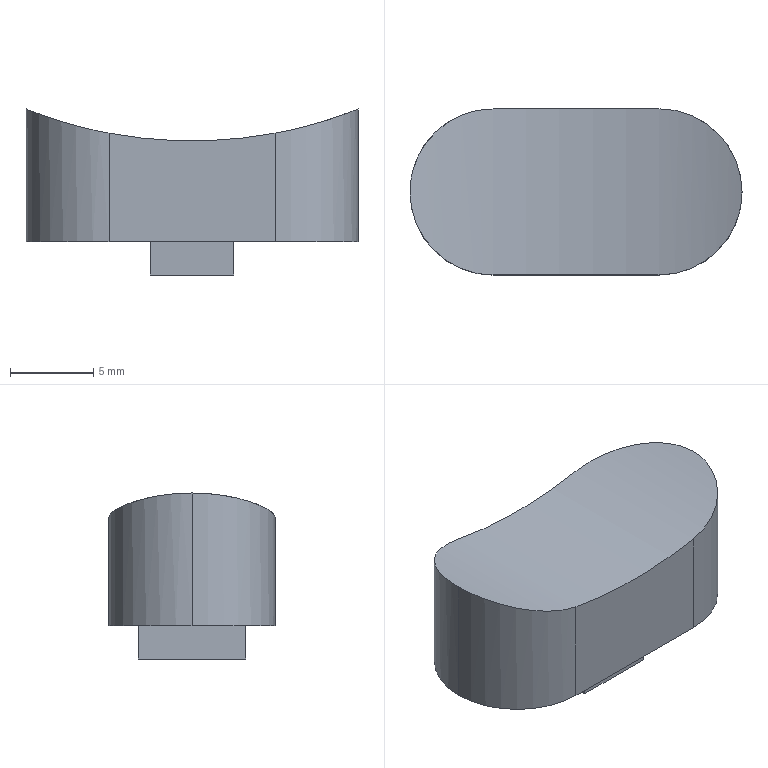Component | SolidWorks | 1UnitDrawer-1_DrawerPanelCloseButton-1 | 1 solid | 16 faces | box 20 x 10 x 10 mm | volume 1218 mm3 | plane 9 | cylinder 7 | commonest cylinder face diameters 10 x4 4 x2 53.852 x1
STEP:
#1=CARTESIAN_POINT('',(-69.695,-8.295,16.457));
#2=VERTEX_POINT('',#1);
#3=CARTESIAN_POINT('',(-69.695,-8.138,16.457));
#4=VERTEX_POINT('',#3);
#5=CARTESIAN_POINT('',(-69.695,-8.216,16.457));
#6=DIRECTION('',(0.,-0.,-1.));
#7=DIRECTION('',(0.,1.,0.));
#8=AXIS2_PLACEMENT_3D('',#5,#6,#7);
#9=CIRCLE('',#8,0.07874);
#10=EDGE_CURVE('',#2,#4,#9,.T.);
#11=ORIENTED_EDGE('',*,*,#10,.T.);
#12=CARTESIAN_POINT('',(-69.695,-8.138,16.535));
#13=VERTEX_POINT('',#12);
#14=CARTESIAN_POINT('',(-69.695,-8.138,16.457));
#15=DIRECTION('',(-0.,0.,1.));
#16=VECTOR('',#15,39.37);
#17=LINE('',#14,#16);
#18=EDGE_CURVE('',#4,#13,#17,.T.);
#19=ORIENTED_EDGE('',*,*,#18,.T.);
#20=CARTESIAN_POINT('',(-69.695,-8.295,16.535));
#21=VERTEX_POINT('',#20);
#22=CARTESIAN_POINT('',(-69.695,-8.216,16.535));
#23=DIRECTION('',(0.,-0.,-1.));
#24=DIRECTION('',(0.,1.,0.));
#25=AXIS2_PLACEMENT_3D('',#22,#23,#24);
#26=CIRCLE('',#25,0.07874);
#27=EDGE_CURVE('',#21,#13,#26,.T.);
#28=ORIENTED_EDGE('',*,*,#27,.F.);
#29=CARTESIAN_POINT('',(-69.695,-8.295,16.457));
#30=DIRECTION('',(-0.,0.,1.));
#31=VECTOR('',#30,39.37);
#32=LINE('',#29,#31);
#33=EDGE_CURVE('',#2,#21,#32,.T.);
#34=ORIENTED_EDGE('',*,*,#33,.F.);
#35=EDGE_LOOP('',(#11,#19,#28,#34));
#36=FACE_OUTER_BOUND('',#35,.T.);
#37=CARTESIAN_POINT('',(-69.695,-8.216,16.457));
#38=DIRECTION('',(-0.,0.,1.));
#39=DIRECTION('',(0.,-1.,0.));
#40=AXIS2_PLACEMENT_3D('',#37,#38,#39);
#41=CYLINDRICAL_SURFACE('',#40,0.07874);
#42=ADVANCED_FACE('',(#36),#41,.F.);
#43=CARTESIAN_POINT('',(-69.891,-8.019,16.535));
#44=VERTEX_POINT('',#43);
#45=CARTESIAN_POINT('',(-69.498,-8.019,16.535));
#46=VERTEX_POINT('',#45);
#47=CARTESIAN_POINT('',(-69.301,-8.019,16.535));
#48=DIRECTION('',(1.,0.,0.));
#49=VECTOR('',#48,39.37);
#50=LINE('',#47,#49);
#51=EDGE_CURVE('',#44,#46,#50,.T.);
#52=ORIENTED_EDGE('',*,*,#51,.T.);
#53=CARTESIAN_POINT('',(-69.301,-8.216,16.535));
#54=VERTEX_POINT('',#53);
#55=CARTESIAN_POINT('',(-69.498,-8.216,16.535));
#56=DIRECTION('',(0.,-0.,-1.));
#57=DIRECTION('',(0.,-1.,0.));
#58=AXIS2_PLACEMENT_3D('',#55,#56,#57);
#59=CIRCLE('',#58,0.1969);
#60=EDGE_CURVE('',#46,#54,#59,.T.);
#61=ORIENTED_EDGE('',*,*,#60,.T.);
#62=CARTESIAN_POINT('',(-69.498,-8.413,16.535));
#63=VERTEX_POINT('',#62);
#64=CARTESIAN_POINT('',(-69.498,-8.216,16.535));
#65=DIRECTION('',(0.,-0.,-1.));
#66=DIRECTION('',(0.,-1.,0.));
#67=AXIS2_PLACEMENT_3D('',#64,#65,#66);
#68=CIRCLE('',#67,0.1969);
#69=EDGE_CURVE('',#54,#63,#68,.T.);
#70=ORIENTED_EDGE('',*,*,#69,.T.);
#71=CARTESIAN_POINT('',(-69.891,-8.413,16.535));
#72=VERTEX_POINT('',#71);
#73=CARTESIAN_POINT('',(-69.301,-8.413,16.535));
#74=DIRECTION('',(1.,0.,0.));
#75=VECTOR('',#74,39.37);
#76=LINE('',#73,#75);
#77=EDGE_CURVE('',#72,#63,#76,.T.);
#78=ORIENTED_EDGE('',*,*,#77,.F.);
#79=CARTESIAN_POINT('',(-70.088,-8.216,16.535));
#80=VERTEX_POINT('',#79);
#81=CARTESIAN_POINT('',(-69.891,-8.216,16.535));
#82=DIRECTION('',(0.,-0.,-1.));
#83=DIRECTION('',(0.,-1.,0.));
#84=AXIS2_PLACEMENT_3D('',#81,#82,#83);
#85=CIRCLE('',#84,0.1969);
#86=EDGE_CURVE('',#72,#80,#85,.T.);
#87=ORIENTED_EDGE('',*,*,#86,.T.);
#88=CARTESIAN_POINT('',(-69.891,-8.216,16.535));
#89=DIRECTION('',(0.,-0.,-1.));
#90=DIRECTION('',(0.,-1.,0.));
#91=AXIS2_PLACEMENT_3D('',#88,#89,#90);
#92=CIRCLE('',#91,0.1969);
#93=EDGE_CURVE('',#80,#44,#92,.T.);
#94=ORIENTED_EDGE('',*,*,#93,.T.);
#95=EDGE_LOOP('',(#52,#61,#70,#78,#87,#94));
#96=FACE_OUTER_BOUND('',#95,.T.);
#97=CARTESIAN_POINT('',(-69.596,-8.088,16.535));
#98=VERTEX_POINT('',#97);
#99=CARTESIAN_POINT('',(-69.596,-8.344,16.535));
#100=VERTEX_POINT('',#99);
#101=CARTESIAN_POINT('',(-69.596,-8.088,16.535));
#102=DIRECTION('',(0.,-1.,0.));
#103=VECTOR('',#102,39.37);
#104=LINE('',#101,#103);
#105=EDGE_CURVE('',#98,#100,#104,.T.);
#106=ORIENTED_EDGE('',*,*,#105,.F.);
#107=CARTESIAN_POINT('',(-69.793,-8.088,16.535));
#108=VERTEX_POINT('',#107);
#109=CARTESIAN_POINT('',(-69.793,-8.088,16.535));
#110=DIRECTION('',(1.,0.,0.));
#111=VECTOR('',#110,39.37);
#112=LINE('',#109,#111);
#113=EDGE_CURVE('',#108,#98,#112,.T.);
#114=ORIENTED_EDGE('',*,*,#113,.F.);
#115=CARTESIAN_POINT('',(-69.793,-8.344,16.535));
#116=VERTEX_POINT('',#115);
#117=CARTESIAN_POINT('',(-69.793,-8.088,16.535));
#118=DIRECTION('',(-0.,1.,-0.));
#119=VECTOR('',#118,39.37);
#120=LINE('',#117,#119);
#121=EDGE_CURVE('',#116,#108,#120,.T.);
#122=ORIENTED_EDGE('',*,*,#121,.F.);
#123=CARTESIAN_POINT('',(-69.793,-8.344,16.535));
#124=DIRECTION('',(-1.,-0.,-0.));
#125=VECTOR('',#124,39.37);
#126=LINE('',#123,#125);
#127=EDGE_CURVE('',#100,#116,#126,.T.);
#128=ORIENTED_EDGE('',*,*,#127,.F.);
#129=EDGE_LOOP('',(#106,#114,#122,#128));
#130=FACE_BOUND('',#129,.T.);
#131=CARTESIAN_POINT('',(-69.301,-8.413,16.535));
#132=DIRECTION('',(-0.,0.,1.));
#133=DIRECTION('',(0.,-1.,0.));
#134=AXIS2_PLACEMENT_3D('',#131,#132,#133);
#135=PLANE('',#134);
#136=ADVANCED_FACE('',(#96,#130),#135,.F.);
#137=CARTESIAN_POINT('',(-69.498,-8.413,16.793));
#138=VERTEX_POINT('',#137);
#139=CARTESIAN_POINT('',(-69.301,-8.216,16.85));
#140=VERTEX_POINT('',#139);
#141=CARTESIAN_POINT('',(-69.498,-8.413,16.793));
#142=CARTESIAN_POINT('',(-69.485,-8.413,16.795));
#143=CARTESIAN_POINT('',(-69.472,-8.412,16.798));
#144=CARTESIAN_POINT('',(-69.453,-8.408,16.802));
#145=CARTESIAN_POINT('',(-69.447,-8.407,16.804));
#146=CARTESIAN_POINT('',(-69.435,-8.403,16.807));
#147=CARTESIAN_POINT('',(-69.429,-8.401,16.808));
#148=CARTESIAN_POINT('',(-69.411,-8.393,16.813));
#149=CARTESIAN_POINT('',(-69.4,-8.387,16.816));
#150=CARTESIAN_POINT('',(-69.378,-8.373,16.823));
#151=CARTESIAN_POINT('',(-69.368,-8.365,16.826));
#152=CARTESIAN_POINT('',(-69.35,-8.347,16.832));
#153=CARTESIAN_POINT('',(-69.342,-8.338,16.835));
#154=CARTESIAN_POINT('',(-69.331,-8.322,16.839));
#155=CARTESIAN_POINT('',(-69.328,-8.316,16.84));
#156=CARTESIAN_POINT('',(-69.322,-8.305,16.842));
#157=CARTESIAN_POINT('',(-69.319,-8.299,16.843));
#158=CARTESIAN_POINT('',(-69.311,-8.281,16.846));
#159=CARTESIAN_POINT('',(-69.307,-8.269,16.848));
#160=CARTESIAN_POINT('',(-69.302,-8.243,16.85));
#161=CARTESIAN_POINT('',(-69.301,-8.23,16.85));
#162=CARTESIAN_POINT('',(-69.301,-8.216,16.85));
#163=B_SPLINE_CURVE_WITH_KNOTS('',3,(#141,#142,#143,#144,#145,#146,#147,#148,#149,#150,#151,#152,#153,#154,#155,#156,#157,#158,#159,#160,#161,#162),.UNSPECIFIED.,.F.,.F.,(4,2,2,2,2,2,2,2,2,2,4),(0.,0.0009953,0.001493,0.001991,0.002986,0.003981,0.004977,0.005474,0.005972,0.006967,0.007963),.UNSPECIFIED.);
#164=EDGE_CURVE('',#138,#140,#163,.T.);
#165=ORIENTED_EDGE('',*,*,#164,.T.);
#166=CARTESIAN_POINT('',(-69.498,-8.019,16.793));
#167=VERTEX_POINT('',#166);
#168=CARTESIAN_POINT('',(-69.301,-8.216,16.85));
#169=CARTESIAN_POINT('',(-69.301,-8.203,16.85));
#170=CARTESIAN_POINT('',(-69.302,-8.19,16.85));
#171=CARTESIAN_POINT('',(-69.307,-8.164,16.848));
#172=CARTESIAN_POINT('',(-69.311,-8.152,16.846));
#173=CARTESIAN_POINT('',(-69.321,-8.128,16.842));
#174=CARTESIAN_POINT('',(-69.327,-8.117,16.84));
#175=CARTESIAN_POINT('',(-69.342,-8.095,16.835));
#176=CARTESIAN_POINT('',(-69.35,-8.085,16.832));
#177=CARTESIAN_POINT('',(-69.368,-8.067,16.826));
#178=CARTESIAN_POINT('',(-69.378,-8.059,16.823));
#179=CARTESIAN_POINT('',(-69.4,-8.045,16.816));
#180=CARTESIAN_POINT('',(-69.411,-8.039,16.813));
#181=CARTESIAN_POINT('',(-69.434,-8.029,16.807));
#182=CARTESIAN_POINT('',(-69.447,-8.026,16.804));
#183=CARTESIAN_POINT('',(-69.472,-8.021,16.798));
#184=CARTESIAN_POINT('',(-69.485,-8.019,16.795));
#185=CARTESIAN_POINT('',(-69.498,-8.019,16.793));
#186=B_SPLINE_CURVE_WITH_KNOTS('',3,(#168,#169,#170,#171,#172,#173,#174,#175,#176,#177,#178,#179,#180,#181,#182,#183,#184,#185),.UNSPECIFIED.,.F.,.F.,(4,2,2,2,2,2,2,2,4),(0.,0.0009953,0.001991,0.002986,0.003981,0.004977,0.005972,0.006967,0.007963),.UNSPECIFIED.);
#187=EDGE_CURVE('',#140,#167,#186,.T.);
#188=ORIENTED_EDGE('',*,*,#187,.T.);
#189=CARTESIAN_POINT('',(-69.891,-8.019,16.793));
#190=VERTEX_POINT('',#189);
#191=CARTESIAN_POINT('',(-69.695,-8.019,17.835));
#192=DIRECTION('',(-0.,1.,-0.));
#193=DIRECTION('',(-1.,-0.,0.));
#194=AXIS2_PLACEMENT_3D('',#191,#192,#193);
#195=CIRCLE('',#194,1.06);
#196=EDGE_CURVE('',#167,#190,#195,.T.);
#197=ORIENTED_EDGE('',*,*,#196,.T.);
#198=CARTESIAN_POINT('',(-70.088,-8.216,16.85));
#199=VERTEX_POINT('',#198);
#200=CARTESIAN_POINT('',(-69.891,-8.019,16.793));
#201=CARTESIAN_POINT('',(-69.904,-8.019,16.795));
#202=CARTESIAN_POINT('',(-69.917,-8.021,16.798));
#203=CARTESIAN_POINT('',(-69.936,-8.024,16.802));
#204=CARTESIAN_POINT('',(-69.942,-8.026,16.804));
#205=CARTESIAN_POINT('',(-69.954,-8.03,16.807));
#206=CARTESIAN_POINT('',(-69.96,-8.032,16.808));
#207=CARTESIAN_POINT('',(-69.978,-8.039,16.813));
#208=CARTESIAN_POINT('',(-69.989,-8.045,16.816));
#209=CARTESIAN_POINT('',(-70.011,-8.059,16.823));
#210=CARTESIAN_POINT('',(-70.021,-8.067,16.826));
#211=CARTESIAN_POINT('',(-70.039,-8.085,16.832));
#212=CARTESIAN_POINT('',(-70.047,-8.095,16.835));
#213=CARTESIAN_POINT('',(-70.058,-8.111,16.839));
#214=CARTESIAN_POINT('',(-70.061,-8.117,16.84));
#215=CARTESIAN_POINT('',(-70.067,-8.128,16.842));
#216=CARTESIAN_POINT('',(-70.07,-8.134,16.843));
#217=CARTESIAN_POINT('',(-70.078,-8.152,16.846));
#218=CARTESIAN_POINT('',(-70.082,-8.164,16.848));
#219=CARTESIAN_POINT('',(-70.087,-8.19,16.85));
#220=CARTESIAN_POINT('',(-70.088,-8.203,16.85));
#221=CARTESIAN_POINT('',(-70.088,-8.216,16.85));
#222=B_SPLINE_CURVE_WITH_KNOTS('',3,(#200,#201,#202,#203,#204,#205,#206,#207,#208,#209,#210,#211,#212,#213,#214,#215,#216,#217,#218,#219,#220,#221),.UNSPECIFIED.,.F.,.F.,(4,2,2,2,2,2,2,2,2,2,4),(0.,0.0009953,0.001493,0.001991,0.002986,0.003981,0.004977,0.005474,0.005972,0.006967,0.007963),.UNSPECIFIED.);
#223=EDGE_CURVE('',#190,#199,#222,.T.);
#224=ORIENTED_EDGE('',*,*,#223,.T.);
#225=CARTESIAN_POINT('',(-69.891,-8.413,16.793));
#226=VERTEX_POINT('',#225);
#227=CARTESIAN_POINT('',(-70.088,-8.216,16.85));
#228=CARTESIAN_POINT('',(-70.088,-8.23,16.85));
#229=CARTESIAN_POINT('',(-70.087,-8.243,16.85));
#230=CARTESIAN_POINT('',(-70.082,-8.268,16.848));
#231=CARTESIAN_POINT('',(-70.078,-8.281,16.846));
#232=CARTESIAN_POINT('',(-70.068,-8.305,16.842));
#233=CARTESIAN_POINT('',(-70.062,-8.316,16.84));
#234=CARTESIAN_POINT('',(-70.047,-8.337,16.835));
#235=CARTESIAN_POINT('',(-70.039,-8.347,16.832));
#236=CARTESIAN_POINT('',(-70.021,-8.365,16.826));
#237=CARTESIAN_POINT('',(-70.011,-8.373,16.823));
#238=CARTESIAN_POINT('',(-69.989,-8.387,16.816));
#239=CARTESIAN_POINT('',(-69.978,-8.393,16.813));
#240=CARTESIAN_POINT('',(-69.955,-8.403,16.807));
#241=CARTESIAN_POINT('',(-69.942,-8.407,16.804));
#242=CARTESIAN_POINT('',(-69.917,-8.412,16.798));
#243=CARTESIAN_POINT('',(-69.904,-8.413,16.795));
#244=CARTESIAN_POINT('',(-69.891,-8.413,16.793));
#245=B_SPLINE_CURVE_WITH_KNOTS('',3,(#227,#228,#229,#230,#231,#232,#233,#234,#235,#236,#237,#238,#239,#240,#241,#242,#243,#244),.UNSPECIFIED.,.F.,.F.,(4,2,2,2,2,2,2,2,4),(0.,0.0009953,0.001991,0.002986,0.003981,0.004977,0.005972,0.006967,0.007963),.UNSPECIFIED.);
#246=EDGE_CURVE('',#199,#226,#245,.T.);
#247=ORIENTED_EDGE('',*,*,#246,.T.);
#248=CARTESIAN_POINT('',(-69.695,-8.413,17.835));
#249=DIRECTION('',(-0.,1.,-0.));
#250=DIRECTION('',(-1.,-0.,0.));
#251=AXIS2_PLACEMENT_3D('',#248,#249,#250);
#252=CIRCLE('',#251,1.06);
#253=EDGE_CURVE('',#138,#226,#252,.T.);
#254=ORIENTED_EDGE('',*,*,#253,.F.);
#255=EDGE_LOOP('',(#165,#188,#197,#224,#247,#254));
#256=FACE_OUTER_BOUND('',#255,.T.);
#257=CARTESIAN_POINT('',(-69.695,-8.413,17.835));
#258=DIRECTION('',(-0.,1.,-0.));
#259=DIRECTION('',(-1.,-0.,0.));
#260=AXIS2_PLACEMENT_3D('',#257,#258,#259);
#261=CYLINDRICAL_SURFACE('',#260,1.06);
#262=ADVANCED_FACE('',(#256),#261,.F.);
#263=ORIENTED_EDGE('',*,*,#77,.T.);
#264=CARTESIAN_POINT('',(-69.498,-8.413,17.835));
#265=DIRECTION('',(-0.,0.,1.));
#266=VECTOR('',#265,39.37);
#267=LINE('',#264,#266);
#268=EDGE_CURVE('',#63,#138,#267,.T.);
#269=ORIENTED_EDGE('',*,*,#268,.T.);
#270=ORIENTED_EDGE('',*,*,#253,.T.);
#271=CARTESIAN_POINT('',(-69.891,-8.413,17.835));
#272=DIRECTION('',(0.,-0.,-1.));
#273=VECTOR('',#272,39.37);
#274=LINE('',#271,#273);
#275=EDGE_CURVE('',#226,#72,#274,.T.);
#276=ORIENTED_EDGE('',*,*,#275,.T.);
#277=EDGE_LOOP('',(#263,#269,#270,#276));
#278=FACE_OUTER_BOUND('',#277,.T.);
#279=CARTESIAN_POINT('',(-69.695,-8.413,17.835));
#280=DIRECTION('',(-0.,1.,-0.));
#281=DIRECTION('',(-1.,-0.,-0.));
#282=AXIS2_PLACEMENT_3D('',#279,#280,#281);
#283=PLANE('',#282);
#284=ADVANCED_FACE('',(#278),#283,.F.);
#285=ORIENTED_EDGE('',*,*,#196,.F.);
#286=CARTESIAN_POINT('',(-69.498,-8.019,16.535));
#287=DIRECTION('',(0.,-0.,-1.));
#288=VECTOR('',#287,39.37);
#289=LINE('',#286,#288);
#290=EDGE_CURVE('',#167,#46,#289,.T.);
#291=ORIENTED_EDGE('',*,*,#290,.T.);
#292=ORIENTED_EDGE('',*,*,#51,.F.);
#293=CARTESIAN_POINT('',(-69.891,-8.019,16.85));
#294=DIRECTION('',(-0.,0.,1.));
#295=VECTOR('',#294,39.37);
#296=LINE('',#293,#295);
#297=EDGE_CURVE('',#44,#190,#296,.T.);
#298=ORIENTED_EDGE('',*,*,#297,.T.);
#299=EDGE_LOOP('',(#285,#291,#292,#298));
#300=FACE_OUTER_BOUND('',#299,.T.);
#301=CARTESIAN_POINT('',(-69.695,-8.019,17.835));
#302=DIRECTION('',(-0.,1.,-0.));
#303=DIRECTION('',(-1.,-0.,-0.));
#304=AXIS2_PLACEMENT_3D('',#301,#302,#303);
#305=PLANE('',#304);
#306=ADVANCED_FACE('',(#300),#305,.T.);
#307=ORIENTED_EDGE('',*,*,#268,.F.);
#308=ORIENTED_EDGE('',*,*,#69,.F.);
#309=CARTESIAN_POINT('',(-69.301,-8.216,16.535));
#310=DIRECTION('',(0.,-0.,-1.));
#311=VECTOR('',#310,39.37);
#312=LINE('',#309,#311);
#313=EDGE_CURVE('',#140,#54,#312,.T.);
#314=ORIENTED_EDGE('',*,*,#313,.F.);
#315=ORIENTED_EDGE('',*,*,#164,.F.);
#316=EDGE_LOOP('',(#307,#308,#314,#315));
#317=FACE_OUTER_BOUND('',#316,.T.);
#318=CARTESIAN_POINT('',(-69.498,-8.216,17.835));
#319=DIRECTION('',(-0.,0.,1.));
#320=DIRECTION('',(0.,-1.,0.));
#321=AXIS2_PLACEMENT_3D('',#318,#319,#320);
#322=CYLINDRICAL_SURFACE('',#321,0.1969);
#323=ADVANCED_FACE('',(#317),#322,.T.);
#324=ORIENTED_EDGE('',*,*,#60,.F.);
#325=ORIENTED_EDGE('',*,*,#290,.F.);
#326=ORIENTED_EDGE('',*,*,#187,.F.);
#327=ORIENTED_EDGE('',*,*,#313,.T.);
#328=EDGE_LOOP('',(#324,#325,#326,#327));
#329=FACE_OUTER_BOUND('',#328,.T.);
#330=CARTESIAN_POINT('',(-69.498,-8.216,16.535));
#331=DIRECTION('',(0.,-0.,-1.));
#332=DIRECTION('',(0.,1.,-0.));
#333=AXIS2_PLACEMENT_3D('',#330,#331,#332);
#334=CYLINDRICAL_SURFACE('',#333,0.1969);
#335=ADVANCED_FACE('',(#329),#334,.T.);
#336=CARTESIAN_POINT('',(-70.088,-8.216,16.535));
#337=DIRECTION('',(0.,-0.,-1.));
#338=VECTOR('',#337,39.37);
#339=LINE('',#336,#338);
#340=EDGE_CURVE('',#199,#80,#339,.T.);
#341=ORIENTED_EDGE('',*,*,#340,.F.);
#342=ORIENTED_EDGE('',*,*,#223,.F.);
#343=ORIENTED_EDGE('',*,*,#297,.F.);
#344=ORIENTED_EDGE('',*,*,#93,.F.);
#345=EDGE_LOOP('',(#341,#342,#343,#344));
#346=FACE_OUTER_BOUND('',#345,.T.);
#347=CARTESIAN_POINT('',(-69.891,-8.216,16.535));
#348=DIRECTION('',(-0.,0.,1.));
#349=DIRECTION('',(0.,-1.,0.));
#350=AXIS2_PLACEMENT_3D('',#347,#348,#349);
#351=CYLINDRICAL_SURFACE('',#350,0.1969);
#352=ADVANCED_FACE('',(#346),#351,.T.);
#353=ORIENTED_EDGE('',*,*,#246,.F.);
#354=ORIENTED_EDGE('',*,*,#340,.T.);
#355=ORIENTED_EDGE('',*,*,#86,.F.);
#356=ORIENTED_EDGE('',*,*,#275,.F.);
#357=EDGE_LOOP('',(#353,#354,#355,#356));
#358=FACE_OUTER_BOUND('',#357,.T.);
#359=CARTESIAN_POINT('',(-69.891,-8.216,17.835));
#360=DIRECTION('',(0.,-0.,-1.));
#361=DIRECTION('',(0.,1.,-0.));
#362=AXIS2_PLACEMENT_3D('',#359,#360,#361);
#363=CYLINDRICAL_SURFACE('',#362,0.1969);
#364=ADVANCED_FACE('',(#358),#363,.T.);
#365=CARTESIAN_POINT('',(-69.596,-8.088,16.457));
#366=VERTEX_POINT('',#365);
#367=CARTESIAN_POINT('',(-69.596,-8.344,16.457));
#368=VERTEX_POINT('',#367);
#369=CARTESIAN_POINT('',(-69.596,-8.088,16.457));
#370=DIRECTION('',(0.,-1.,0.));
#371=VECTOR('',#370,39.37);
#372=LINE('',#369,#371);
#373=EDGE_CURVE('',#366,#368,#372,.T.);
#374=ORIENTED_EDGE('',*,*,#373,.T.);
#375=CARTESIAN_POINT('',(-69.793,-8.344,16.457));
#376=VERTEX_POINT('',#375);
#377=CARTESIAN_POINT('',(-69.793,-8.344,16.457));
#378=DIRECTION('',(-1.,-0.,-0.));
#379=VECTOR('',#378,39.37);
#380=LINE('',#377,#379);
#381=EDGE_CURVE('',#368,#376,#380,.T.);
#382=ORIENTED_EDGE('',*,*,#381,.T.);
#383=CARTESIAN_POINT('',(-69.793,-8.088,16.457));
#384=VERTEX_POINT('',#383);
#385=CARTESIAN_POINT('',(-69.793,-8.088,16.457));
#386=DIRECTION('',(-0.,1.,-0.));
#387=VECTOR('',#386,39.37);
#388=LINE('',#385,#387);
#389=EDGE_CURVE('',#376,#384,#388,.T.);
#390=ORIENTED_EDGE('',*,*,#389,.T.);
#391=CARTESIAN_POINT('',(-69.793,-8.088,16.457));
#392=DIRECTION('',(1.,0.,0.));
#393=VECTOR('',#392,39.37);
#394=LINE('',#391,#393);
#395=EDGE_CURVE('',#384,#366,#394,.T.);
#396=ORIENTED_EDGE('',*,*,#395,.T.);
#397=EDGE_LOOP('',(#374,#382,#390,#396));
#398=FACE_OUTER_BOUND('',#397,.T.);
#399=ORIENTED_EDGE('',*,*,#10,.F.);
#400=CARTESIAN_POINT('',(-69.695,-8.216,16.457));
#401=DIRECTION('',(0.,-0.,-1.));
#402=DIRECTION('',(0.,1.,0.));
#403=AXIS2_PLACEMENT_3D('',#400,#401,#402);
#404=CIRCLE('',#403,0.07874);
#405=EDGE_CURVE('',#4,#2,#404,.T.);
#406=ORIENTED_EDGE('',*,*,#405,.F.);
#407=EDGE_LOOP('',(#399,#406));
#408=FACE_BOUND('',#407,.T.);
#409=CARTESIAN_POINT('',(-69.596,-8.344,16.457));
#410=DIRECTION('',(-0.,0.,1.));
#411=DIRECTION('',(0.,-1.,0.));
#412=AXIS2_PLACEMENT_3D('',#409,#410,#411);
#413=PLANE('',#412);
#414=ADVANCED_FACE('',(#398,#408),#413,.F.);
#415=ORIENTED_EDGE('',*,*,#105,.T.);
#416=CARTESIAN_POINT('',(-69.596,-8.344,16.457));
#417=DIRECTION('',(-0.,0.,1.));
#418=VECTOR('',#417,39.37);
#419=LINE('',#416,#418);
#420=EDGE_CURVE('',#368,#100,#419,.T.);
#421=ORIENTED_EDGE('',*,*,#420,.F.);
#422=ORIENTED_EDGE('',*,*,#373,.F.);
#423=CARTESIAN_POINT('',(-69.596,-8.088,16.457));
#424=DIRECTION('',(-0.,0.,1.));
#425=VECTOR('',#424,39.37);
#426=LINE('',#423,#425);
#427=EDGE_CURVE('',#366,#98,#426,.T.);
#428=ORIENTED_EDGE('',*,*,#427,.T.);
#429=EDGE_LOOP('',(#415,#421,#422,#428));
#430=FACE_OUTER_BOUND('',#429,.T.);
#431=CARTESIAN_POINT('',(-69.596,-8.088,16.457));
#432=DIRECTION('',(-1.,-0.,-0.));
#433=DIRECTION('',(0.,-1.,0.));
#434=AXIS2_PLACEMENT_3D('',#431,#432,#433);
#435=PLANE('',#434);
#436=ADVANCED_FACE('',(#430),#435,.F.);
#437=ORIENTED_EDGE('',*,*,#127,.T.);
#438=CARTESIAN_POINT('',(-69.793,-8.344,16.457));
#439=DIRECTION('',(-0.,0.,1.));
#440=VECTOR('',#439,39.37);
#441=LINE('',#438,#440);
#442=EDGE_CURVE('',#376,#116,#441,.T.);
#443=ORIENTED_EDGE('',*,*,#442,.F.);
#444=ORIENTED_EDGE('',*,*,#381,.F.);
#445=ORIENTED_EDGE('',*,*,#420,.T.);
#446=EDGE_LOOP('',(#437,#443,#444,#445));
#447=FACE_OUTER_BOUND('',#446,.T.);
#448=CARTESIAN_POINT('',(-69.793,-8.344,16.457));
#449=DIRECTION('',(-0.,1.,-0.));
#450=DIRECTION('',(-1.,-0.,-0.));
#451=AXIS2_PLACEMENT_3D('',#448,#449,#450);
#452=PLANE('',#451);
#453=ADVANCED_FACE('',(#447),#452,.F.);
#454=ORIENTED_EDGE('',*,*,#121,.T.);
#455=CARTESIAN_POINT('',(-69.793,-8.088,16.457));
#456=DIRECTION('',(-0.,0.,1.));
#457=VECTOR('',#456,39.37);
#458=LINE('',#455,#457);
#459=EDGE_CURVE('',#384,#108,#458,.T.);
#460=ORIENTED_EDGE('',*,*,#459,.F.);
#461=ORIENTED_EDGE('',*,*,#389,.F.);
#462=ORIENTED_EDGE('',*,*,#442,.T.);
#463=EDGE_LOOP('',(#454,#460,#461,#462));
#464=FACE_OUTER_BOUND('',#463,.T.);
#465=CARTESIAN_POINT('',(-69.793,-8.088,16.457));
#466=DIRECTION('',(1.,0.,0.));
#467=DIRECTION('',(-0.,1.,-0.));
#468=AXIS2_PLACEMENT_3D('',#465,#466,#467);
#469=PLANE('',#468);
#470=ADVANCED_FACE('',(#464),#469,.F.);
#471=ORIENTED_EDGE('',*,*,#113,.T.);
#472=ORIENTED_EDGE('',*,*,#427,.F.);
#473=ORIENTED_EDGE('',*,*,#395,.F.);
#474=ORIENTED_EDGE('',*,*,#459,.T.);
#475=EDGE_LOOP('',(#471,#472,#473,#474));
#476=FACE_OUTER_BOUND('',#475,.T.);
#477=CARTESIAN_POINT('',(-69.793,-8.088,16.457));
#478=DIRECTION('',(0.,-1.,0.));
#479=DIRECTION('',(1.,0.,0.));
#480=AXIS2_PLACEMENT_3D('',#477,#478,#479);
#481=PLANE('',#480);
#482=ADVANCED_FACE('',(#476),#481,.F.);
#483=ORIENTED_EDGE('',*,*,#18,.F.);
#484=ORIENTED_EDGE('',*,*,#405,.T.);
#485=ORIENTED_EDGE('',*,*,#33,.T.);
#486=CARTESIAN_POINT('',(-69.695,-8.216,16.535));
#487=DIRECTION('',(0.,-0.,-1.));
#488=DIRECTION('',(0.,1.,0.));
#489=AXIS2_PLACEMENT_3D('',#486,#487,#488);
#490=CIRCLE('',#489,0.07874);
#491=EDGE_CURVE('',#13,#21,#490,.T.);
#492=ORIENTED_EDGE('',*,*,#491,.F.);
#493=EDGE_LOOP('',(#483,#484,#485,#492));
#494=FACE_OUTER_BOUND('',#493,.T.);
#495=CARTESIAN_POINT('',(-69.695,-8.216,16.457));
#496=DIRECTION('',(-0.,0.,1.));
#497=DIRECTION('',(0.,-1.,0.));
#498=AXIS2_PLACEMENT_3D('',#495,#496,#497);
#499=CYLINDRICAL_SURFACE('',#498,0.07874);
#500=ADVANCED_FACE('',(#494),#499,.F.);
#501=ORIENTED_EDGE('',*,*,#27,.T.);
#502=ORIENTED_EDGE('',*,*,#491,.T.);
#503=EDGE_LOOP('',(#501,#502));
#504=FACE_OUTER_BOUND('',#503,.T.);
#505=CARTESIAN_POINT('',(-69.301,-8.413,16.535));
#506=DIRECTION('',(-0.,0.,1.));
#507=DIRECTION('',(0.,-1.,0.));
#508=AXIS2_PLACEMENT_3D('',#505,#506,#507);
#509=PLANE('',#508);
#510=ADVANCED_FACE('',(#504),#509,.F.);
#511=CLOSED_SHELL('',(#42,#136,#262,#284,#306,#323,#335,#352,#364,#414,#436,#453,#470,#482,#500,#510));
#512=MANIFOLD_SOLID_BREP('',#511);
#513=CARTESIAN_POINT('',(0.,0.,0.));
#514=DIRECTION('',(0.,0.,1.));
#515=DIRECTION('',(1.,0.,0.));
#516=AXIS2_PLACEMENT_3D('',#513,#514,#515);
#517=(LENGTH_UNIT()NAMED_UNIT(*)SI_UNIT($,.METRE.));
#518=LENGTH_MEASURE_WITH_UNIT(LENGTH_MEASURE(0.0254),#517);
#519=DIMENSIONAL_EXPONENTS(1.,0.,0.,0.,0.,0.,0.);
#520=(CONVERSION_BASED_UNIT('',#518)LENGTH_UNIT()NAMED_UNIT(#519));
#521=UNCERTAINTY_MEASURE_WITH_UNIT(LENGTH_MEASURE(0.00001),#520,'','');
#522=(NAMED_UNIT(*)PLANE_ANGLE_UNIT()SI_UNIT($,.RADIAN.));
#523=(NAMED_UNIT(*)SI_UNIT($,.STERADIAN.)SOLID_ANGLE_UNIT());
#524=(GEOMETRIC_REPRESENTATION_CONTEXT(3)GLOBAL_UNCERTAINTY_ASSIGNED_CONTEXT((#521))GLOBAL_UNIT_ASSIGNED_CONTEXT((#520,#522,#523))REPRESENTATION_CONTEXT('',''));
#525=ADVANCED_BREP_SHAPE_REPRESENTATION('',(#512,#516),#524);
#526=COLOUR_RGB('',0.7922,0.8196,0.9333);
#527=FILL_AREA_STYLE_COLOUR('',#526);
#528=FILL_AREA_STYLE('',(#527));
#529=SURFACE_STYLE_FILL_AREA(#528);
#530=SURFACE_SIDE_STYLE('',(#529));
#531=SURFACE_STYLE_USAGE(.BOTH.,#530);
#532=PRESENTATION_STYLE_ASSIGNMENT((#531));
#533=STYLED_ITEM('',(#532),#512);
#534=PRESENTATION_LAYER_ASSIGNMENT('','',(#533));
#535=(LENGTH_UNIT()NAMED_UNIT(*)SI_UNIT($,.METRE.));
#536=LENGTH_MEASURE_WITH_UNIT(LENGTH_MEASURE(0.0254),#535);
#537=DIMENSIONAL_EXPONENTS(1.,0.,0.,0.,0.,0.,0.);
#538=(CONVERSION_BASED_UNIT('',#536)LENGTH_UNIT()NAMED_UNIT(#537));
#539=UNCERTAINTY_MEASURE_WITH_UNIT(LENGTH_MEASURE(0.00001),#538,'','');
#540=(NAMED_UNIT(*)PLANE_ANGLE_UNIT()SI_UNIT($,.RADIAN.));
#541=(NAMED_UNIT(*)SI_UNIT($,.STERADIAN.)SOLID_ANGLE_UNIT());
#542=(GEOMETRIC_REPRESENTATION_CONTEXT(3)GLOBAL_UNCERTAINTY_ASSIGNED_CONTEXT((#539))GLOBAL_UNIT_ASSIGNED_CONTEXT((#538,#540,#541))REPRESENTATION_CONTEXT('',''));
#543=MECHANICAL_DESIGN_GEOMETRIC_PRESENTATION_REPRESENTATION('',(#533),#542);